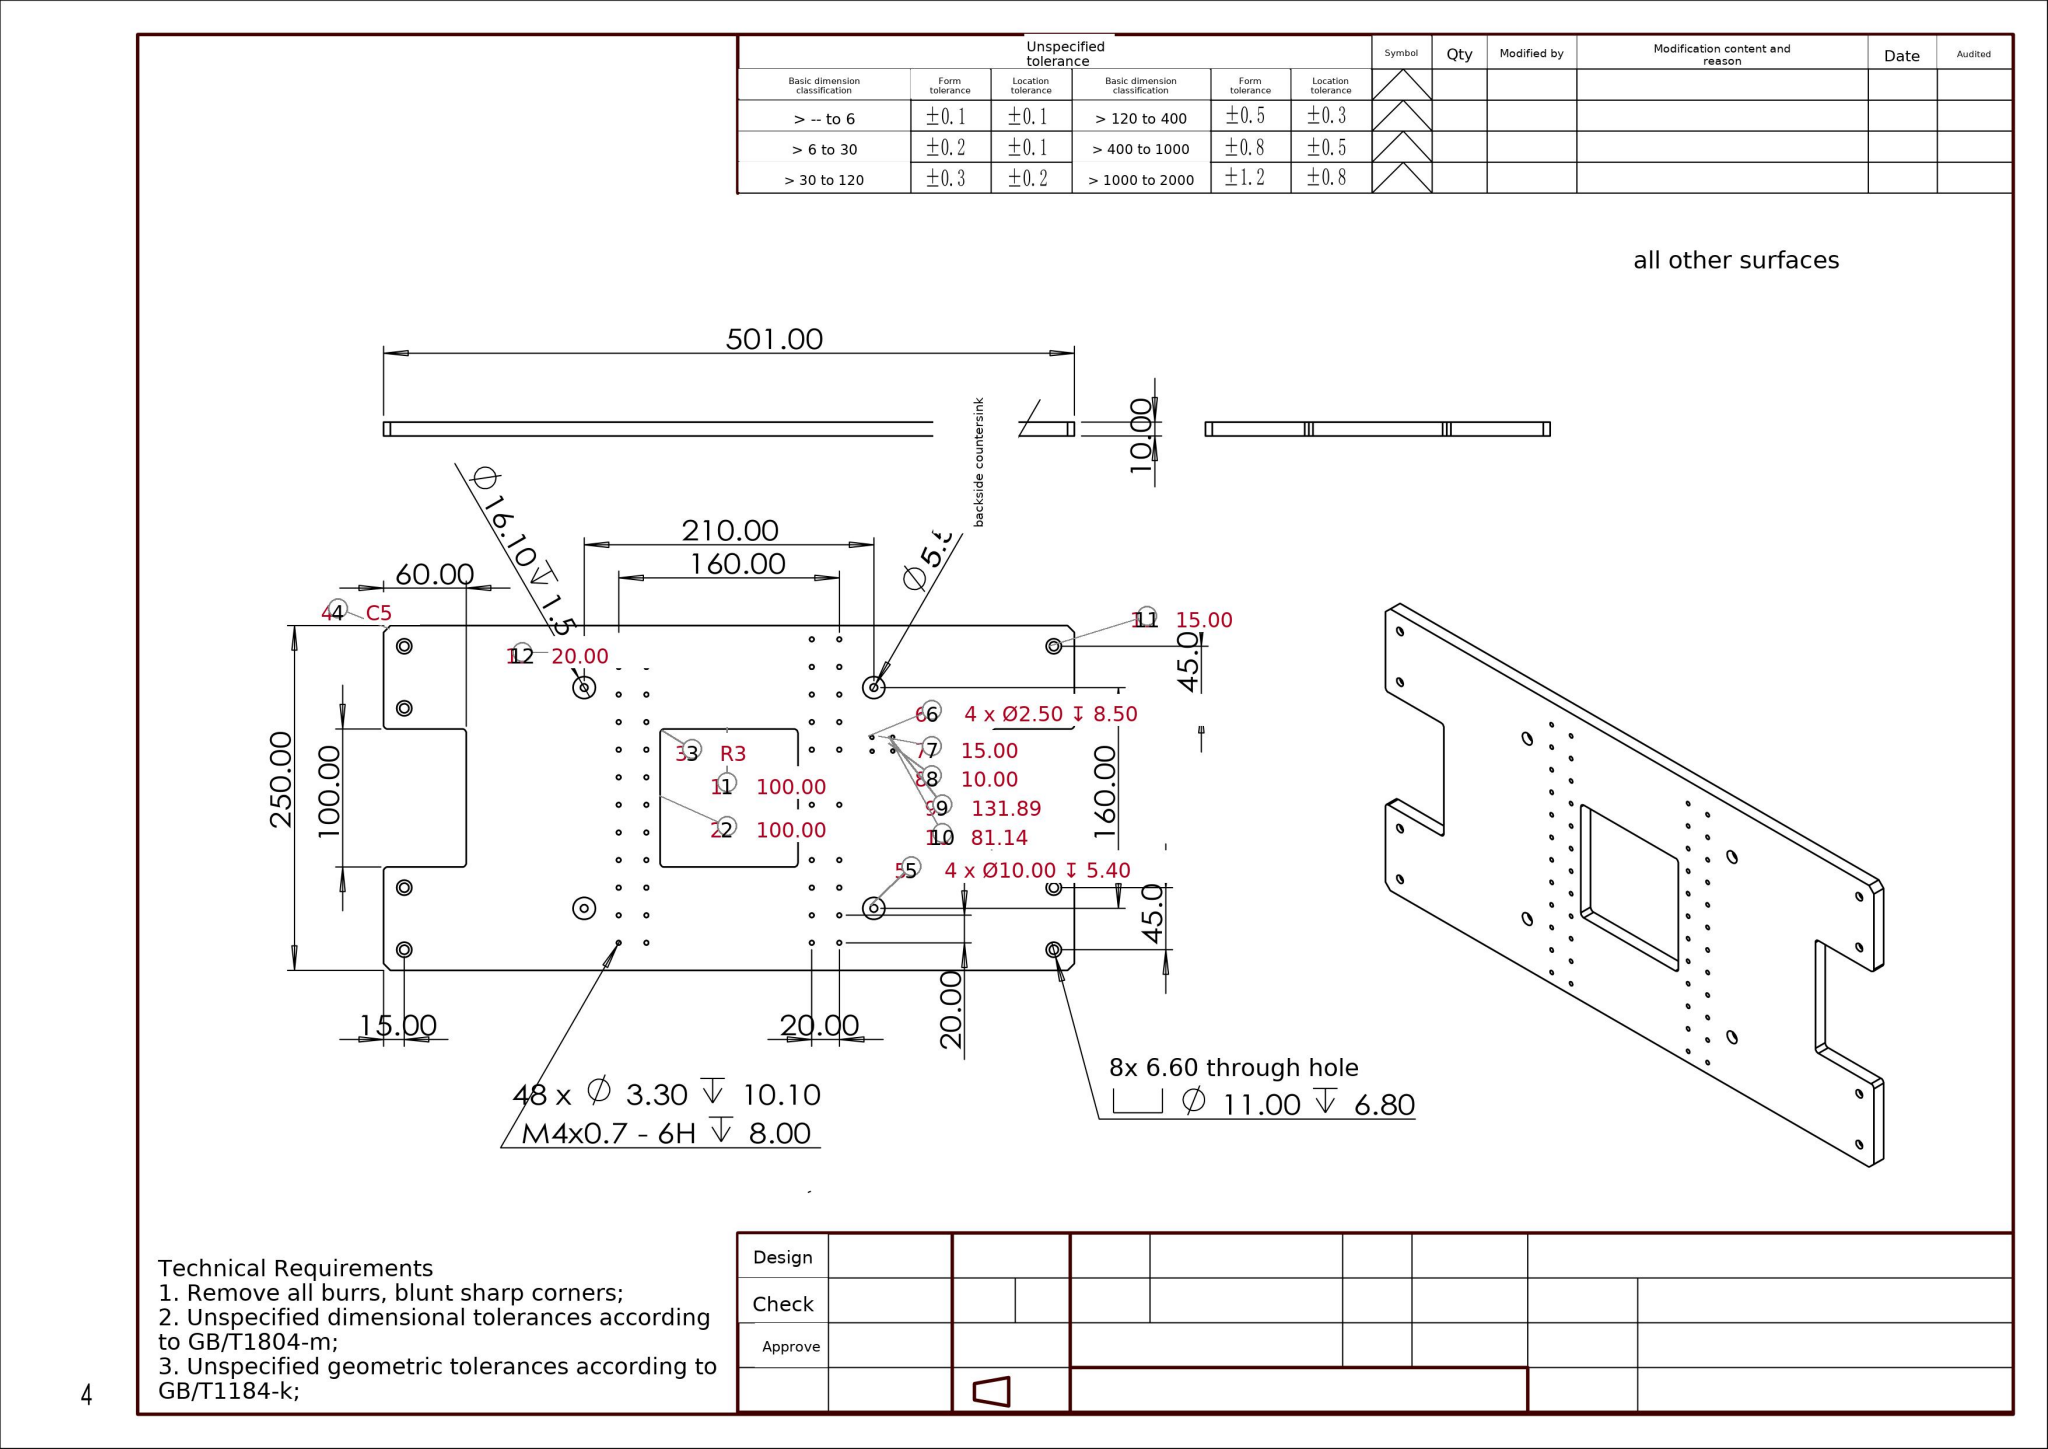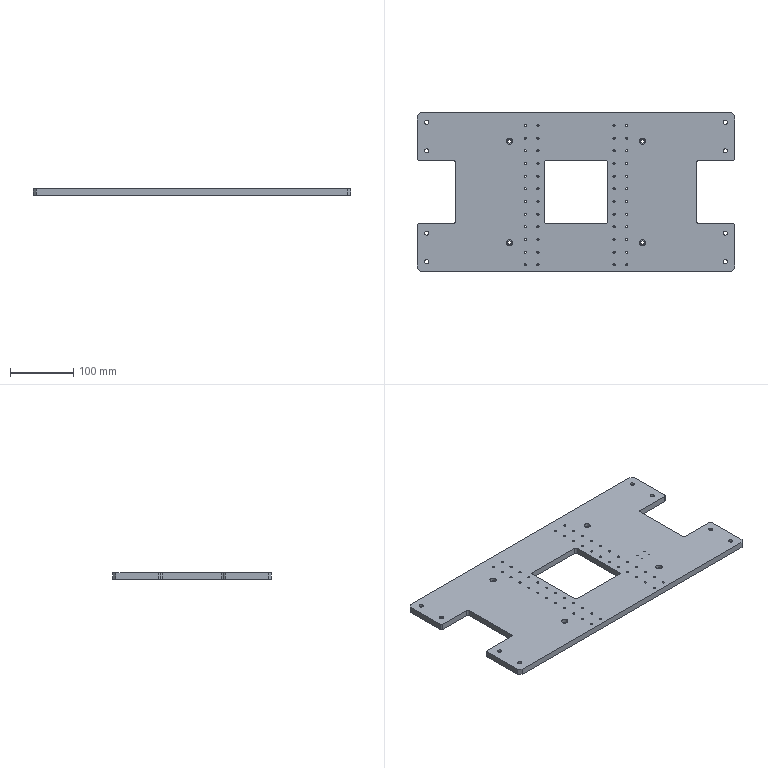Part | SolidWorks | mm | 1 solid | 218 faces | box 501 x 250 x 10 mm | volume 1018542 mm3 | cylinder 172 | plane 38 | cone 8 | commonest cylinder face diameters 3.3 x96 11 x16 6.6 x16 6 x12 2.5 x8 16.1 x8 10 x8 5.5 x8
build123d program:
from build123d import *

# Parameters (mm, degrees)
SKETCH1_W                                         = 501
SKETCH1_H                                         = 250
BOSS_EXTRUDE1_DEPTH                               = 10
M5_HEX_SOCKET_HEAD_CAP_SCREW_CBORE1_D             = 5.5
M5_HEX_SOCKET_HEAD_CAP_SCREW_CBORE1_CBORE_D       = 10
M5_HEX_SOCKET_HEAD_CAP_SCREW_CBORE1_CBORE_DEPTH   = 5.4
SKETCH11_R                                        = 8.05
CUT_EXTRUDE4_DEPTH                                = 1.5
CHAMFER1_SIZE                                     = 5
M3_TAPPED_HOLE1_D                                 = 2.5
M3_TAPPED_HOLE1_DEPTH                             = 8.5
M3_TAPPED_HOLE1_TIP                               = 0.7511
SKETCH14_W                                        = 120
SKETCH14_H                                        = 100
CUT_EXTRUDE5_DEPTH                                = 10
SKETCH15_W                                        = 100
SKETCH15_H                                        = 100
CUT_EXTRUDE6_DEPTH                                = 10
HOLE_SIZE_ACCORDING_TO_HEXAGON_SOCKET_D           = 6.6
HOLE_SIZE_ACCORDING_TO_HEXAGON_SOCKET_CBORE_D     = 11
HOLE_SIZE_ACCORDING_TO_HEXAGON_SOCKET_CBORE_DEPTH = 6.8
FILLET1_R                                         = 3
M4X0_7_TAPPED_HOLE1_AT_2_COUNT                    = 2
M4X0_7_TAPPED_HOLE1_AT_2_PITCH                    = 20
M4X0_7_TAPPED_HOLE1_AT_3_COUNT                    = 2
M4X0_7_TAPPED_HOLE1_AT_3_PITCH                    = 20
M4X0_7_TAPPED_HOLE1_AT_4_COUNT                    = 2
M4X0_7_TAPPED_HOLE1_AT_4_PITCH                    = 28.284
M4X0_7_TAPPED_HOLE1_AT_5_COUNT                    = 2
M4X0_7_TAPPED_HOLE1_AT_5_PITCH                    = 40
M4X0_7_TAPPED_HOLE1_AT_6_COUNT                    = 2
M4X0_7_TAPPED_HOLE1_AT_6_PITCH                    = 44.721
M4X0_7_TAPPED_HOLE1_AT_7_COUNT                    = 2
M4X0_7_TAPPED_HOLE1_AT_7_PITCH                    = 60
M4X0_7_TAPPED_HOLE1_AT_8_COUNT                    = 2
M4X0_7_TAPPED_HOLE1_AT_8_PITCH                    = 63.246
M4X0_7_TAPPED_HOLE1_AT_9_COUNT                    = 2
M4X0_7_TAPPED_HOLE1_AT_9_PITCH                    = 80
M4X0_7_TAPPED_HOLE1_AT_10_COUNT                   = 2
M4X0_7_TAPPED_HOLE1_AT_10_PITCH                   = 82.462
M4X0_7_TAPPED_HOLE1_AT_11_COUNT                   = 2
M4X0_7_TAPPED_HOLE1_AT_11_PITCH                   = 100
M4X0_7_TAPPED_HOLE1_AT_12_COUNT                   = 2
M4X0_7_TAPPED_HOLE1_AT_12_PITCH                   = 101.98
M4X0_7_TAPPED_HOLE1_AT_13_COUNT                   = 2
M4X0_7_TAPPED_HOLE1_AT_13_PITCH                   = 120
M4X0_7_TAPPED_HOLE1_AT_14_COUNT                   = 2
M4X0_7_TAPPED_HOLE1_AT_14_PITCH                   = 121.655
M4X0_7_TAPPED_HOLE1_AT_15_COUNT                   = 2
M4X0_7_TAPPED_HOLE1_AT_15_PITCH                   = 140
M4X0_7_TAPPED_HOLE1_AT_16_COUNT                   = 2
M4X0_7_TAPPED_HOLE1_AT_16_PITCH                   = 141.421
M4X0_7_TAPPED_HOLE1_AT_17_COUNT                   = 2
M4X0_7_TAPPED_HOLE1_AT_17_PITCH                   = 160
M4X0_7_TAPPED_HOLE1_AT_18_COUNT                   = 2
M4X0_7_TAPPED_HOLE1_AT_18_PITCH                   = 161.245
M4X0_7_TAPPED_HOLE1_AT_19_COUNT                   = 2
M4X0_7_TAPPED_HOLE1_AT_19_PITCH                   = 180
M4X0_7_TAPPED_HOLE1_AT_20_COUNT                   = 2
M4X0_7_TAPPED_HOLE1_AT_20_PITCH                   = 181.108
M4X0_7_TAPPED_HOLE1_AT_21_COUNT                   = 2
M4X0_7_TAPPED_HOLE1_AT_21_PITCH                   = 200
M4X0_7_TAPPED_HOLE1_AT_22_COUNT                   = 2
M4X0_7_TAPPED_HOLE1_AT_22_PITCH                   = 200.998
M4X0_7_TAPPED_HOLE1_AT_23_COUNT                   = 2
M4X0_7_TAPPED_HOLE1_AT_23_PITCH                   = 220
M4X0_7_TAPPED_HOLE1_AT_24_COUNT                   = 2
M4X0_7_TAPPED_HOLE1_AT_24_PITCH                   = 220.907


with BuildPart() as part:
    # Sketch1 → Boss-Extrude1 (new body)
    with BuildSketch(Plane.XY):
        Rectangle(SKETCH1_W, SKETCH1_H)
    extrude(amount=BOSS_EXTRUDE1_DEPTH)

    # M5 Hex Socket Head Cap Screw CBORE1 (through all)
    with Locations(Plane.XY.offset(10)):
        with Locations((105, 80), (-105, 80), (-105, -80), (105, -80)):
            CounterBoreHole(M5_HEX_SOCKET_HEAD_CAP_SCREW_CBORE1_D / 2, M5_HEX_SOCKET_HEAD_CAP_SCREW_CBORE1_CBORE_D / 2, M5_HEX_SOCKET_HEAD_CAP_SCREW_CBORE1_CBORE_DEPTH)

    # Sketch11 → Cut-Extrude4 (cut)
    with BuildSketch(Plane(origin=(0, 0, 0), x_dir=(-1, 0, 0), z_dir=(0, 0, -1))):
        with Locations((-105, 80)):
            Circle(SKETCH11_R)
        with Locations((105, 80)):
            Circle(SKETCH11_R)
        with Locations((-105, -80)):
            Circle(SKETCH11_R)
        with Locations((105, -80)):
            Circle(SKETCH11_R)
    extrude(amount=-CUT_EXTRUDE4_DEPTH, mode=Mode.SUBTRACT)

    # Chamfer1
    chamfer1_edges = [part.edges().sort_by_distance(p)[0] for p in [
        (250.5, -125, 5),
        (-250.5, -125, 5),
        (-250.5, 125, 5),
        (250.5, 125, 5),
    ]]
    chamfer(chamfer1_edges, length=CHAMFER1_SIZE)

    # M3 Tapped Hole1
    with Locations(Plane(origin=(0, 0, 0), x_dir=(-1, 0, 0), z_dir=(0, 0, -1))):
        with Locations((-118.614, -44.032), (-118.728, -34.033), (-103.729, -33.862), (-103.615, -43.861)):
            Hole(M3_TAPPED_HOLE1_D / 2, depth=M3_TAPPED_HOLE1_DEPTH)
            with Locations((0, 0, -(M3_TAPPED_HOLE1_DEPTH + M3_TAPPED_HOLE1_TIP / 2))):  # 118° drill point
                Cone(0, M3_TAPPED_HOLE1_D / 2, M3_TAPPED_HOLE1_TIP, mode=Mode.SUBTRACT)

    # Sketch14 → Cut-Extrude5 (cut)
    with BuildSketch(Plane.XY.offset(10)):
        with Locations((-250.5, 0)):
            Rectangle(SKETCH14_W, SKETCH14_H)
    cut_extrude5 = extrude(amount=-CUT_EXTRUDE5_DEPTH, mode=Mode.SUBTRACT)

    # Sketch15 → Cut-Extrude6 (cut)
    with BuildSketch(Plane.XY.offset(10)):
        Rectangle(SKETCH15_W, SKETCH15_H)
    extrude(amount=-CUT_EXTRUDE6_DEPTH, mode=Mode.SUBTRACT)

    # Hole Size _ according to_ Hexagon Socket (through all)
    with Locations(Plane(origin=(0, 0, 0), x_dir=(-1, 0, 0), z_dir=(0, 0, -1))):
        with Locations((235.5, 65), (235.5, 110), (235.5, -110), (235.5, -65), (-235.5, -110), (-235.5, -65), (-235.5, 65), (-235.5, 110)):
            CounterBoreHole(HOLE_SIZE_ACCORDING_TO_HEXAGON_SOCKET_D / 2, HOLE_SIZE_ACCORDING_TO_HEXAGON_SOCKET_CBORE_D / 2, HOLE_SIZE_ACCORDING_TO_HEXAGON_SOCKET_CBORE_DEPTH)

    # Mirror2: Cut-Extrude5 across plane
    add(cut_extrude5.mirror(Plane(origin=(0, 0, 0), x_dir=(0, 0, 1), z_dir=(1, 0, 0))), mode=Mode.SUBTRACT)

    # Fillet1
    fillet1_edges = [part.edges().sort_by_distance(p)[0] for p in [
        (-250.5, -50, 5),
        (-190.5, -50, 5),
        (-250.5, 50, 5),
        (-190.5, 50, 5),
        (50, 50, 5),
        (50, -50, 5),
        (-50, -50, 5),
        (-50, 50, 5),
        (190.5, 50, 5),
        (190.5, -50, 5),
        (250.5, 50, 5),
        (250.5, -50, 5),
    ]]
    fillet(fillet1_edges, radius=FILLET1_R)

    # Sketch23 → M4x0.7 Tapped Hole1 (revolve, cut)
    with BuildSketch(Plane(origin=(-60, -115, 10), x_dir=(0, -1, 0), z_dir=(1, 0, 0))):
        Polygon((0, 0), (0, 11.091), (1.65, 10.1), (1.65, 0), align=None)
    m4x0_7_tapped_hole1 = revolve(axis=Axis((-60, -115, 16.35), (0, 0, -1)), mode=Mode.SUBTRACT)

    # M4x0.7 Tapped Hole1 at 2: M4x0.7 Tapped Hole1 ×2
    with Locations(*[(-i * M4X0_7_TAPPED_HOLE1_AT_2_PITCH, 0, 0) for i in range(1, M4X0_7_TAPPED_HOLE1_AT_2_COUNT)]):
        add(m4x0_7_tapped_hole1, mode=Mode.SUBTRACT)

    # M4x0.7 Tapped Hole1 at 3: M4x0.7 Tapped Hole1 ×2
    with Locations(*[(0, i * M4X0_7_TAPPED_HOLE1_AT_3_PITCH, 0) for i in range(1, M4X0_7_TAPPED_HOLE1_AT_3_COUNT)]):
        add(m4x0_7_tapped_hole1, mode=Mode.SUBTRACT)

    # M4x0.7 Tapped Hole1 at 4: M4x0.7 Tapped Hole1 ×2
    with Locations(*[Vector(-0.7071, 0.7071, 0) * (i * M4X0_7_TAPPED_HOLE1_AT_4_PITCH) for i in range(1, M4X0_7_TAPPED_HOLE1_AT_4_COUNT)]):
        add(m4x0_7_tapped_hole1, mode=Mode.SUBTRACT)

    # M4x0.7 Tapped Hole1 at 5: M4x0.7 Tapped Hole1 ×2
    with Locations(*[(0, i * M4X0_7_TAPPED_HOLE1_AT_5_PITCH, 0) for i in range(1, M4X0_7_TAPPED_HOLE1_AT_5_COUNT)]):
        add(m4x0_7_tapped_hole1, mode=Mode.SUBTRACT)

    # M4x0.7 Tapped Hole1 at 6: M4x0.7 Tapped Hole1 ×2
    with Locations(*[Vector(-0.4472, 0.8944, 0) * (i * M4X0_7_TAPPED_HOLE1_AT_6_PITCH) for i in range(1, M4X0_7_TAPPED_HOLE1_AT_6_COUNT)]):
        add(m4x0_7_tapped_hole1, mode=Mode.SUBTRACT)

    # M4x0.7 Tapped Hole1 at 7: M4x0.7 Tapped Hole1 ×2
    with Locations(*[(0, i * M4X0_7_TAPPED_HOLE1_AT_7_PITCH, 0) for i in range(1, M4X0_7_TAPPED_HOLE1_AT_7_COUNT)]):
        add(m4x0_7_tapped_hole1, mode=Mode.SUBTRACT)

    # M4x0.7 Tapped Hole1 at 8: M4x0.7 Tapped Hole1 ×2
    with Locations(*[Vector(-0.3162, 0.9487, 0) * (i * M4X0_7_TAPPED_HOLE1_AT_8_PITCH) for i in range(1, M4X0_7_TAPPED_HOLE1_AT_8_COUNT)]):
        add(m4x0_7_tapped_hole1, mode=Mode.SUBTRACT)

    # M4x0.7 Tapped Hole1 at 9: M4x0.7 Tapped Hole1 ×2
    with Locations(*[(0, i * M4X0_7_TAPPED_HOLE1_AT_9_PITCH, 0) for i in range(1, M4X0_7_TAPPED_HOLE1_AT_9_COUNT)]):
        add(m4x0_7_tapped_hole1, mode=Mode.SUBTRACT)

    # M4x0.7 Tapped Hole1 at 10: M4x0.7 Tapped Hole1 ×2
    with Locations(*[Vector(-0.2425, 0.9701, 0) * (i * M4X0_7_TAPPED_HOLE1_AT_10_PITCH) for i in range(1, M4X0_7_TAPPED_HOLE1_AT_10_COUNT)]):
        add(m4x0_7_tapped_hole1, mode=Mode.SUBTRACT)

    # M4x0.7 Tapped Hole1 at 11: M4x0.7 Tapped Hole1 ×2
    with Locations(*[(0, i * M4X0_7_TAPPED_HOLE1_AT_11_PITCH, 0) for i in range(1, M4X0_7_TAPPED_HOLE1_AT_11_COUNT)]):
        add(m4x0_7_tapped_hole1, mode=Mode.SUBTRACT)

    # M4x0.7 Tapped Hole1 at 12: M4x0.7 Tapped Hole1 ×2
    with Locations(*[Vector(-0.1961, 0.9806, 0) * (i * M4X0_7_TAPPED_HOLE1_AT_12_PITCH) for i in range(1, M4X0_7_TAPPED_HOLE1_AT_12_COUNT)]):
        add(m4x0_7_tapped_hole1, mode=Mode.SUBTRACT)

    # M4x0.7 Tapped Hole1 at 13: M4x0.7 Tapped Hole1 ×2
    with Locations(*[(0, i * M4X0_7_TAPPED_HOLE1_AT_13_PITCH, 0) for i in range(1, M4X0_7_TAPPED_HOLE1_AT_13_COUNT)]):
        add(m4x0_7_tapped_hole1, mode=Mode.SUBTRACT)

    # M4x0.7 Tapped Hole1 at 14: M4x0.7 Tapped Hole1 ×2
    with Locations(*[Vector(-0.1644, 0.9864, 0) * (i * M4X0_7_TAPPED_HOLE1_AT_14_PITCH) for i in range(1, M4X0_7_TAPPED_HOLE1_AT_14_COUNT)]):
        add(m4x0_7_tapped_hole1, mode=Mode.SUBTRACT)

    # M4x0.7 Tapped Hole1 at 15: M4x0.7 Tapped Hole1 ×2
    with Locations(*[(0, i * M4X0_7_TAPPED_HOLE1_AT_15_PITCH, 0) for i in range(1, M4X0_7_TAPPED_HOLE1_AT_15_COUNT)]):
        add(m4x0_7_tapped_hole1, mode=Mode.SUBTRACT)

    # M4x0.7 Tapped Hole1 at 16: M4x0.7 Tapped Hole1 ×2
    with Locations(*[Vector(-0.1414, 0.9899, 0) * (i * M4X0_7_TAPPED_HOLE1_AT_16_PITCH) for i in range(1, M4X0_7_TAPPED_HOLE1_AT_16_COUNT)]):
        add(m4x0_7_tapped_hole1, mode=Mode.SUBTRACT)

    # M4x0.7 Tapped Hole1 at 17: M4x0.7 Tapped Hole1 ×2
    with Locations(*[(0, i * M4X0_7_TAPPED_HOLE1_AT_17_PITCH, 0) for i in range(1, M4X0_7_TAPPED_HOLE1_AT_17_COUNT)]):
        add(m4x0_7_tapped_hole1, mode=Mode.SUBTRACT)

    # M4x0.7 Tapped Hole1 at 18: M4x0.7 Tapped Hole1 ×2
    with Locations(*[Vector(-0.124, 0.9923, 0) * (i * M4X0_7_TAPPED_HOLE1_AT_18_PITCH) for i in range(1, M4X0_7_TAPPED_HOLE1_AT_18_COUNT)]):
        add(m4x0_7_tapped_hole1, mode=Mode.SUBTRACT)

    # M4x0.7 Tapped Hole1 at 19: M4x0.7 Tapped Hole1 ×2
    with Locations(*[(0, i * M4X0_7_TAPPED_HOLE1_AT_19_PITCH, 0) for i in range(1, M4X0_7_TAPPED_HOLE1_AT_19_COUNT)]):
        add(m4x0_7_tapped_hole1, mode=Mode.SUBTRACT)

    # M4x0.7 Tapped Hole1 at 20: M4x0.7 Tapped Hole1 ×2
    with Locations(*[Vector(-0.1104, 0.9939, 0) * (i * M4X0_7_TAPPED_HOLE1_AT_20_PITCH) for i in range(1, M4X0_7_TAPPED_HOLE1_AT_20_COUNT)]):
        add(m4x0_7_tapped_hole1, mode=Mode.SUBTRACT)

    # M4x0.7 Tapped Hole1 at 21: M4x0.7 Tapped Hole1 ×2
    with Locations(*[(0, i * M4X0_7_TAPPED_HOLE1_AT_21_PITCH, 0) for i in range(1, M4X0_7_TAPPED_HOLE1_AT_21_COUNT)]):
        add(m4x0_7_tapped_hole1, mode=Mode.SUBTRACT)

    # M4x0.7 Tapped Hole1 at 22: M4x0.7 Tapped Hole1 ×2
    with Locations(*[Vector(-0.0995, 0.995, 0) * (i * M4X0_7_TAPPED_HOLE1_AT_22_PITCH) for i in range(1, M4X0_7_TAPPED_HOLE1_AT_22_COUNT)]):
        add(m4x0_7_tapped_hole1, mode=Mode.SUBTRACT)

    # M4x0.7 Tapped Hole1 at 23: M4x0.7 Tapped Hole1 ×2
    with Locations(*[(0, i * M4X0_7_TAPPED_HOLE1_AT_23_PITCH, 0) for i in range(1, M4X0_7_TAPPED_HOLE1_AT_23_COUNT)]):
        add(m4x0_7_tapped_hole1, mode=Mode.SUBTRACT)

    # M4x0.7 Tapped Hole1 at 24: M4x0.7 Tapped Hole1 ×2
    with Locations(*[Vector(-0.09054, 0.9959, 0) * (i * M4X0_7_TAPPED_HOLE1_AT_24_PITCH) for i in range(1, M4X0_7_TAPPED_HOLE1_AT_24_COUNT)]):
        add(m4x0_7_tapped_hole1, mode=Mode.SUBTRACT)

    # Mirror3: M4x0.7 Tapped Hole1 across plane
    add(m4x0_7_tapped_hole1.mirror(Plane(origin=(0, 0, 0), x_dir=(0, 0, 1), z_dir=(1, 0, 0))), mode=Mode.SUBTRACT)

    # Mirror3 copy 1 sketch → Mirror3 copy 1 (revolve, cut)
    with BuildSketch(Plane(origin=(80, -115, 10), x_dir=(0, -1, 0), z_dir=(-1, 0, 0))):
        Polygon((0, 0), (0, -11.091), (1.65, -10.1), (1.65, 0), align=None)
    revolve(axis=Axis((80, -115, 16.35), (0, 0, 1)), mode=Mode.SUBTRACT)

    # Mirror3 copy 2 sketch → Mirror3 copy 2 (revolve, cut)
    with BuildSketch(Plane(origin=(60, -95, 10), x_dir=(0, -1, 0), z_dir=(-1, 0, 0))):
        Polygon((0, 0), (0, -11.091), (1.65, -10.1), (1.65, 0), align=None)
    revolve(axis=Axis((60, -95, 16.35), (0, 0, 1)), mode=Mode.SUBTRACT)

    # Mirror3 copy 3 sketch → Mirror3 copy 3 (revolve, cut)
    with BuildSketch(Plane(origin=(80, -95, 10), x_dir=(0, -1, 0), z_dir=(-1, 0, 0))):
        Polygon((0, 0), (0, -11.091), (1.65, -10.1), (1.65, 0), align=None)
    revolve(axis=Axis((80, -95, 16.35), (0, 0, 1)), mode=Mode.SUBTRACT)

    # Mirror3 copy 4 sketch → Mirror3 copy 4 (revolve, cut)
    with BuildSketch(Plane(origin=(60, -75, 10), x_dir=(0, -1, 0), z_dir=(-1, 0, 0))):
        Polygon((0, 0), (0, -11.091), (1.65, -10.1), (1.65, 0), align=None)
    revolve(axis=Axis((60, -75, 16.35), (0, 0, 1)), mode=Mode.SUBTRACT)

    # Mirror3 copy 5 sketch → Mirror3 copy 5 (revolve, cut)
    with BuildSketch(Plane(origin=(80, -75, 10), x_dir=(0, -1, 0), z_dir=(-1, 0, 0))):
        Polygon((0, 0), (0, -11.091), (1.65, -10.1), (1.65, 0), align=None)
    revolve(axis=Axis((80, -75, 16.35), (0, 0, 1)), mode=Mode.SUBTRACT)

    # Mirror3 copy 6 sketch → Mirror3 copy 6 (revolve, cut)
    with BuildSketch(Plane(origin=(60, -55, 10), x_dir=(0, -1, 0), z_dir=(-1, 0, 0))):
        Polygon((0, 0), (0, -11.091), (1.65, -10.1), (1.65, 0), align=None)
    revolve(axis=Axis((60, -55, 16.35), (0, 0, 1)), mode=Mode.SUBTRACT)

    # Mirror3 copy 7 sketch → Mirror3 copy 7 (revolve, cut)
    with BuildSketch(Plane(origin=(80, -55, 10), x_dir=(0, -1, 0), z_dir=(-1, 0, 0))):
        Polygon((0, 0), (0, -11.091), (1.65, -10.1), (1.65, 0), align=None)
    revolve(axis=Axis((80, -55, 16.35), (0, 0, 1)), mode=Mode.SUBTRACT)

    # Mirror3 copy 8 sketch → Mirror3 copy 8 (revolve, cut)
    with BuildSketch(Plane(origin=(60, -35, 10), x_dir=(0, -1, 0), z_dir=(-1, 0, 0))):
        Polygon((0, 0), (0, -11.091), (1.65, -10.1), (1.65, 0), align=None)
    revolve(axis=Axis((60, -35, 16.35), (0, 0, 1)), mode=Mode.SUBTRACT)

    # Mirror3 copy 9 sketch → Mirror3 copy 9 (revolve, cut)
    with BuildSketch(Plane(origin=(80, -35, 10), x_dir=(0, -1, 0), z_dir=(-1, 0, 0))):
        Polygon((0, 0), (0, -11.091), (1.65, -10.1), (1.65, 0), align=None)
    revolve(axis=Axis((80, -35, 16.35), (0, 0, 1)), mode=Mode.SUBTRACT)

    # Mirror3 copy 10 sketch → Mirror3 copy 10 (revolve, cut)
    with BuildSketch(Plane(origin=(60, -15, 10), x_dir=(0, -1, 0), z_dir=(-1, 0, 0))):
        Polygon((0, 0), (0, -11.091), (1.65, -10.1), (1.65, 0), align=None)
    revolve(axis=Axis((60, -15, 16.35), (0, 0, 1)), mode=Mode.SUBTRACT)

    # Mirror3 copy 11 sketch → Mirror3 copy 11 (revolve, cut)
    with BuildSketch(Plane(origin=(80, -15, 10), x_dir=(0, -1, 0), z_dir=(-1, 0, 0))):
        Polygon((0, 0), (0, -11.091), (1.65, -10.1), (1.65, 0), align=None)
    revolve(axis=Axis((80, -15, 16.35), (0, 0, 1)), mode=Mode.SUBTRACT)

    # Mirror3 copy 12 sketch → Mirror3 copy 12 (revolve, cut)
    with BuildSketch(Plane(origin=(60, 5, 10), x_dir=(0, -1, 0), z_dir=(-1, 0, 0))):
        Polygon((0, 0), (0, -11.091), (1.65, -10.1), (1.65, 0), align=None)
    revolve(axis=Axis((60, 5, 16.35), (0, 0, 1)), mode=Mode.SUBTRACT)

    # Mirror3 copy 13 sketch → Mirror3 copy 13 (revolve, cut)
    with BuildSketch(Plane(origin=(80, 5, 10), x_dir=(0, -1, 0), z_dir=(-1, 0, 0))):
        Polygon((0, 0), (0, -11.091), (1.65, -10.1), (1.65, 0), align=None)
    revolve(axis=Axis((80, 5, 16.35), (0, 0, 1)), mode=Mode.SUBTRACT)

    # Mirror3 copy 14 sketch → Mirror3 copy 14 (revolve, cut)
    with BuildSketch(Plane(origin=(60, 25, 10), x_dir=(0, -1, 0), z_dir=(-1, 0, 0))):
        Polygon((0, 0), (0, -11.091), (1.65, -10.1), (1.65, 0), align=None)
    revolve(axis=Axis((60, 25, 16.35), (0, 0, 1)), mode=Mode.SUBTRACT)

    # Mirror3 copy 15 sketch → Mirror3 copy 15 (revolve, cut)
    with BuildSketch(Plane(origin=(80, 25, 10), x_dir=(0, -1, 0), z_dir=(-1, 0, 0))):
        Polygon((0, 0), (0, -11.091), (1.65, -10.1), (1.65, 0), align=None)
    revolve(axis=Axis((80, 25, 16.35), (0, 0, 1)), mode=Mode.SUBTRACT)

    # Mirror3 copy 16 sketch → Mirror3 copy 16 (revolve, cut)
    with BuildSketch(Plane(origin=(60, 45, 10), x_dir=(0, -1, 0), z_dir=(-1, 0, 0))):
        Polygon((0, 0), (0, -11.091), (1.65, -10.1), (1.65, 0), align=None)
    revolve(axis=Axis((60, 45, 16.35), (0, 0, 1)), mode=Mode.SUBTRACT)

    # Mirror3 copy 17 sketch → Mirror3 copy 17 (revolve, cut)
    with BuildSketch(Plane(origin=(80, 45, 10), x_dir=(0, -1, 0), z_dir=(-1, 0, 0))):
        Polygon((0, 0), (0, -11.091), (1.65, -10.1), (1.65, 0), align=None)
    revolve(axis=Axis((80, 45, 16.35), (0, 0, 1)), mode=Mode.SUBTRACT)

    # Mirror3 copy 18 sketch → Mirror3 copy 18 (revolve, cut)
    with BuildSketch(Plane(origin=(60, 65, 10), x_dir=(0, -1, 0), z_dir=(-1, 0, 0))):
        Polygon((0, 0), (0, -11.091), (1.65, -10.1), (1.65, 0), align=None)
    revolve(axis=Axis((60, 65, 16.35), (0, 0, 1)), mode=Mode.SUBTRACT)

    # Mirror3 copy 19 sketch → Mirror3 copy 19 (revolve, cut)
    with BuildSketch(Plane(origin=(80, 65, 10), x_dir=(0, -1, 0), z_dir=(-1, 0, 0))):
        Polygon((0, 0), (0, -11.091), (1.65, -10.1), (1.65, 0), align=None)
    revolve(axis=Axis((80, 65, 16.35), (0, 0, 1)), mode=Mode.SUBTRACT)

    # Mirror3 copy 20 sketch → Mirror3 copy 20 (revolve, cut)
    with BuildSketch(Plane(origin=(60, 85, 10), x_dir=(0, -1, 0), z_dir=(-1, 0, 0))):
        Polygon((0, 0), (0, -11.091), (1.65, -10.1), (1.65, 0), align=None)
    revolve(axis=Axis((60, 85, 16.35), (0, 0, 1)), mode=Mode.SUBTRACT)

    # Mirror3 copy 21 sketch → Mirror3 copy 21 (revolve, cut)
    with BuildSketch(Plane(origin=(80, 85, 10), x_dir=(0, -1, 0), z_dir=(-1, 0, 0))):
        Polygon((0, 0), (0, -11.091), (1.65, -10.1), (1.65, 0), align=None)
    revolve(axis=Axis((80, 85, 16.35), (0, 0, 1)), mode=Mode.SUBTRACT)

    # Mirror3 copy 22 sketch → Mirror3 copy 22 (revolve, cut)
    with BuildSketch(Plane(origin=(60, 105, 10), x_dir=(0, -1, 0), z_dir=(-1, 0, 0))):
        Polygon((0, 0), (0, -11.091), (1.65, -10.1), (1.65, 0), align=None)
    revolve(axis=Axis((60, 105, 16.35), (0, 0, 1)), mode=Mode.SUBTRACT)

    # Mirror3 copy 23 sketch → Mirror3 copy 23 (revolve, cut)
    with BuildSketch(Plane(origin=(80, 105, 10), x_dir=(0, -1, 0), z_dir=(-1, 0, 0))):
        Polygon((0, 0), (0, -11.091), (1.65, -10.1), (1.65, 0), align=None)
    revolve(axis=Axis((80, 105, 16.35), (0, 0, 1)), mode=Mode.SUBTRACT)


solid = part.part